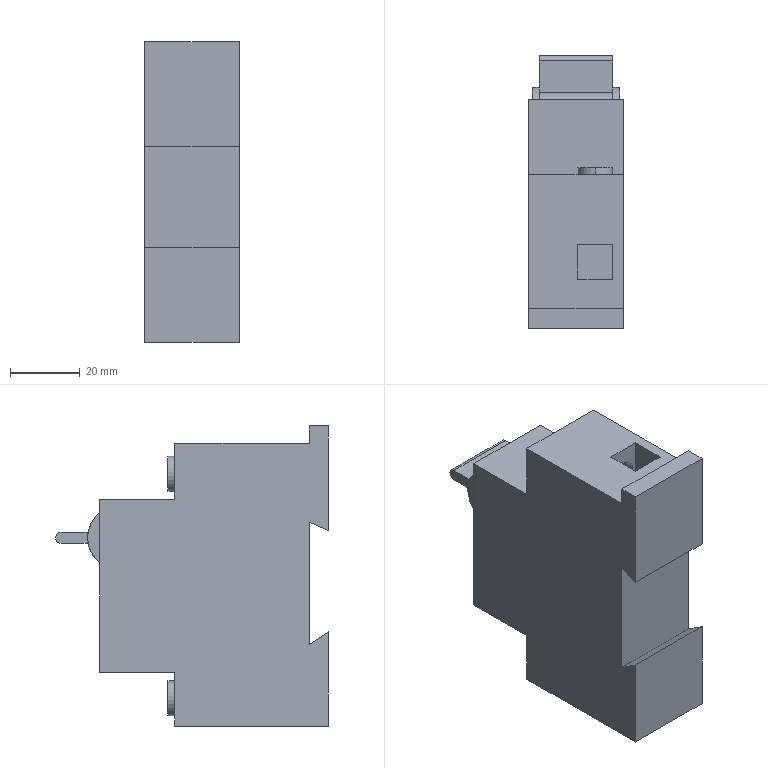Component | SolidWorks | C120HighCurrentMiniatureCircuitBreaker-2 | 1 solid | 61 faces | volume 117337 mm3 | plane 45 | cylinder 16 | commonest cylinder face diameters 10 x4 8 x2 8.049 x2 7.962 x2 3.2 x2 18 x2 15.5 x2